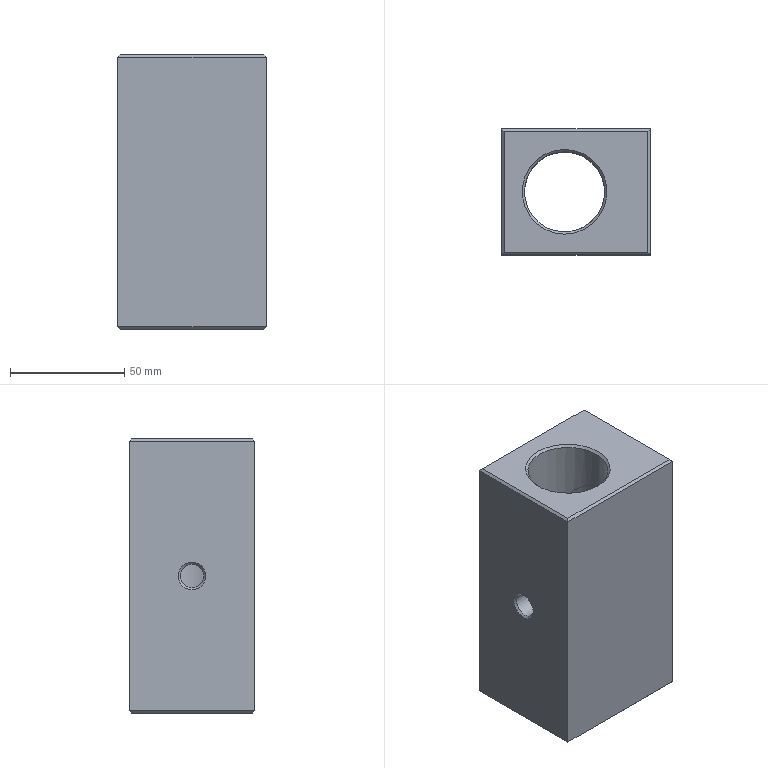Component | NX | YMSR_PET_P03 | 1 solid | 33 faces | volume 309053 mm3 | plane 14 | cone 12 | cylinder 7 | commonest cylinder face diameters 6.8 x4 35.1 x2 10.3 x1